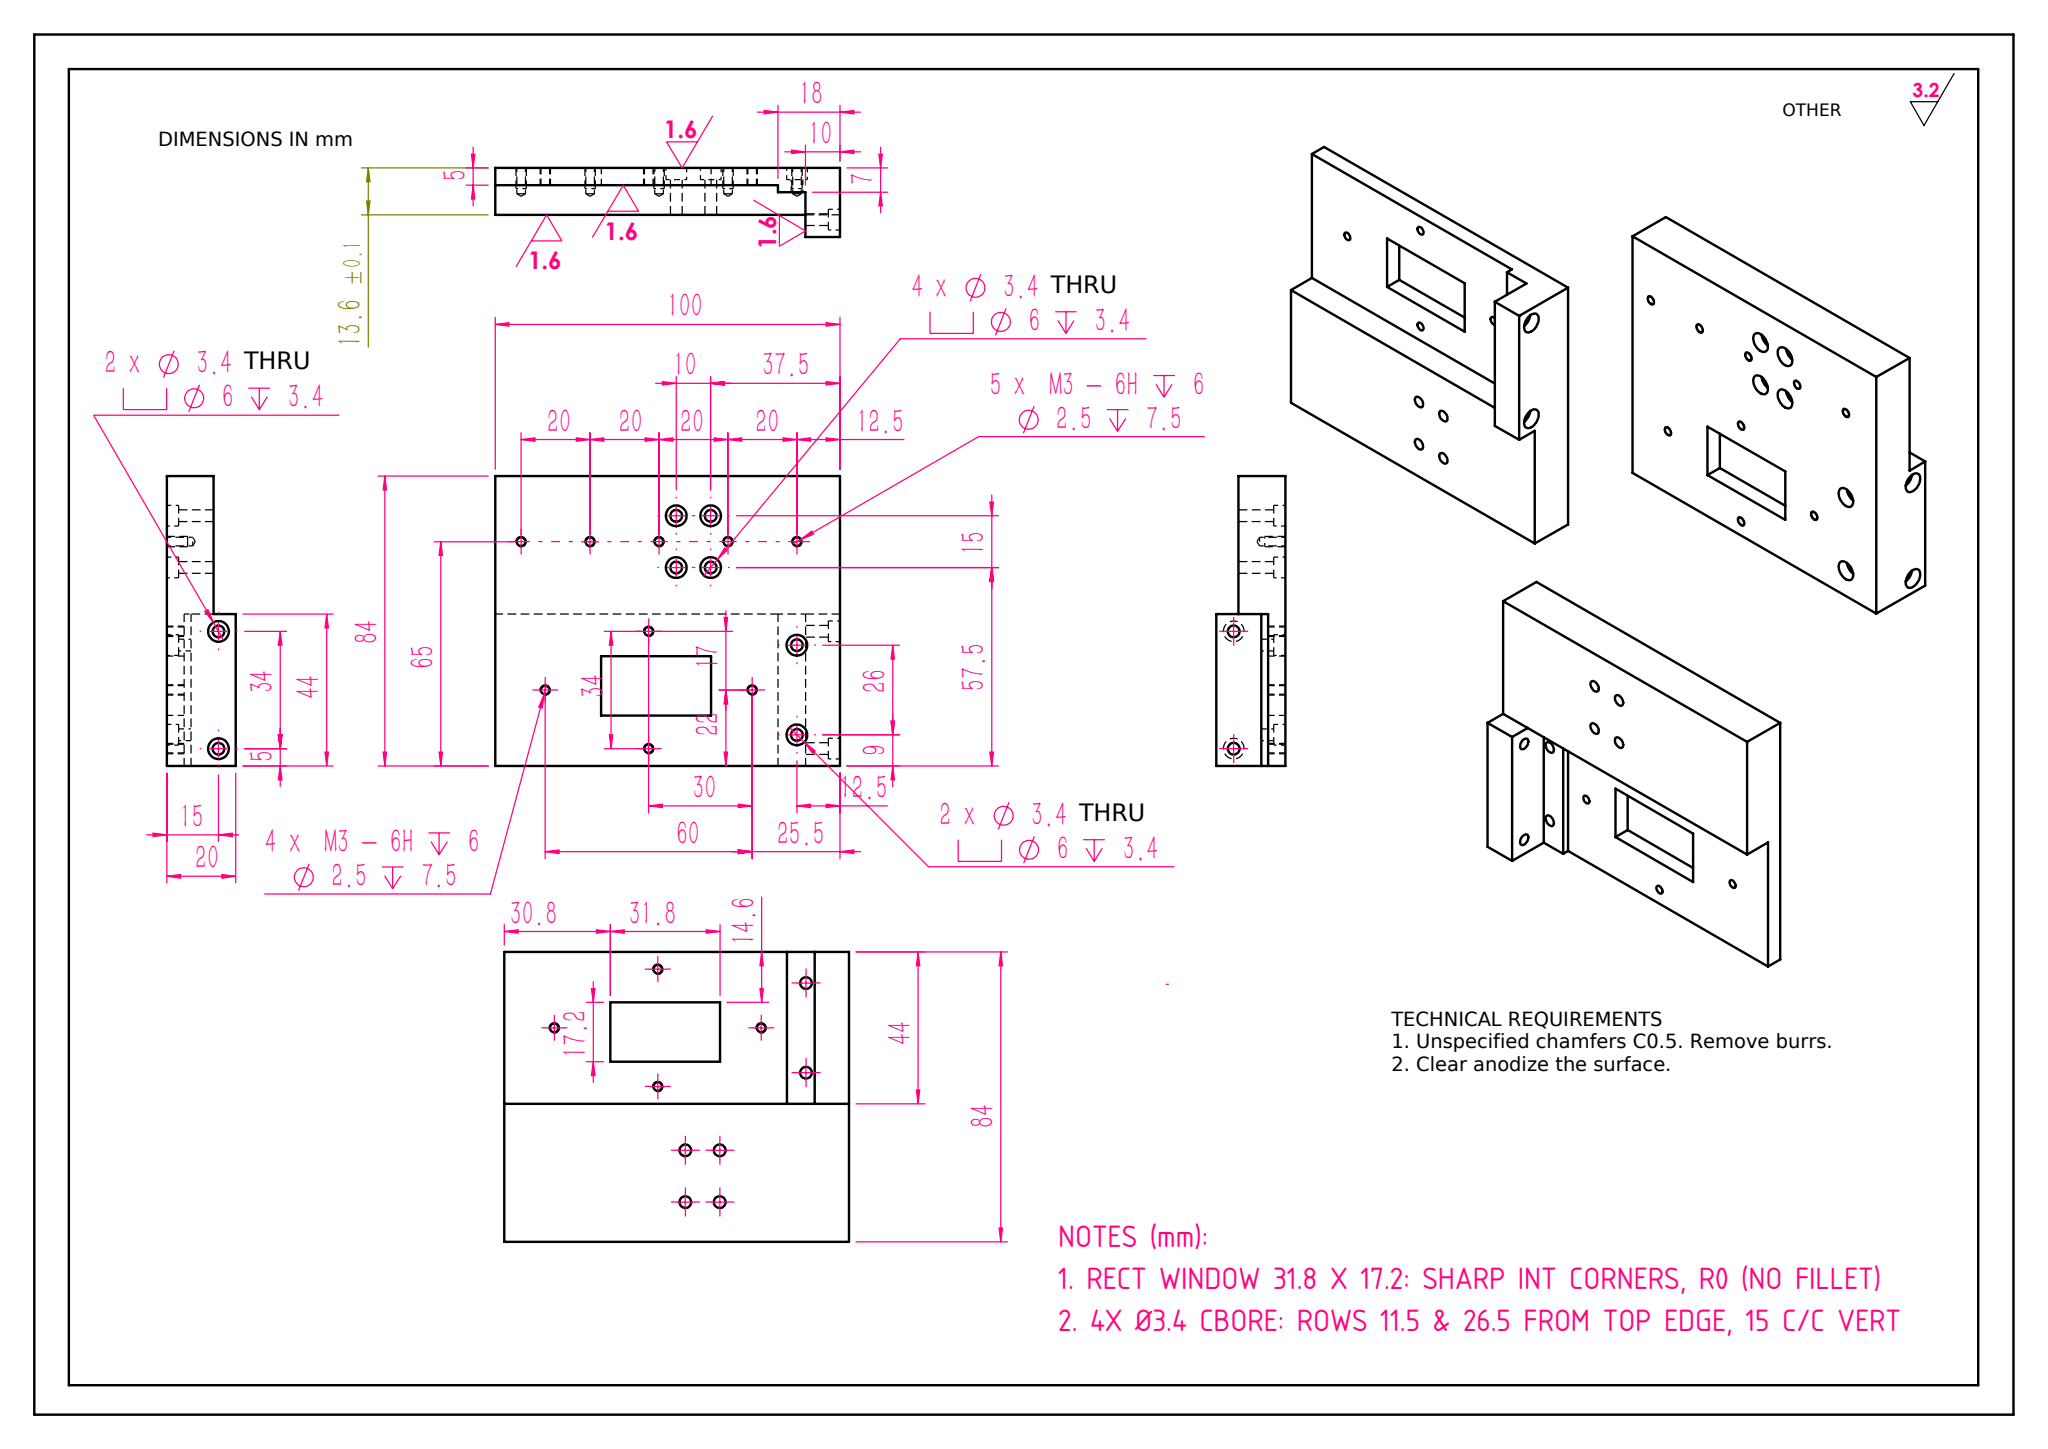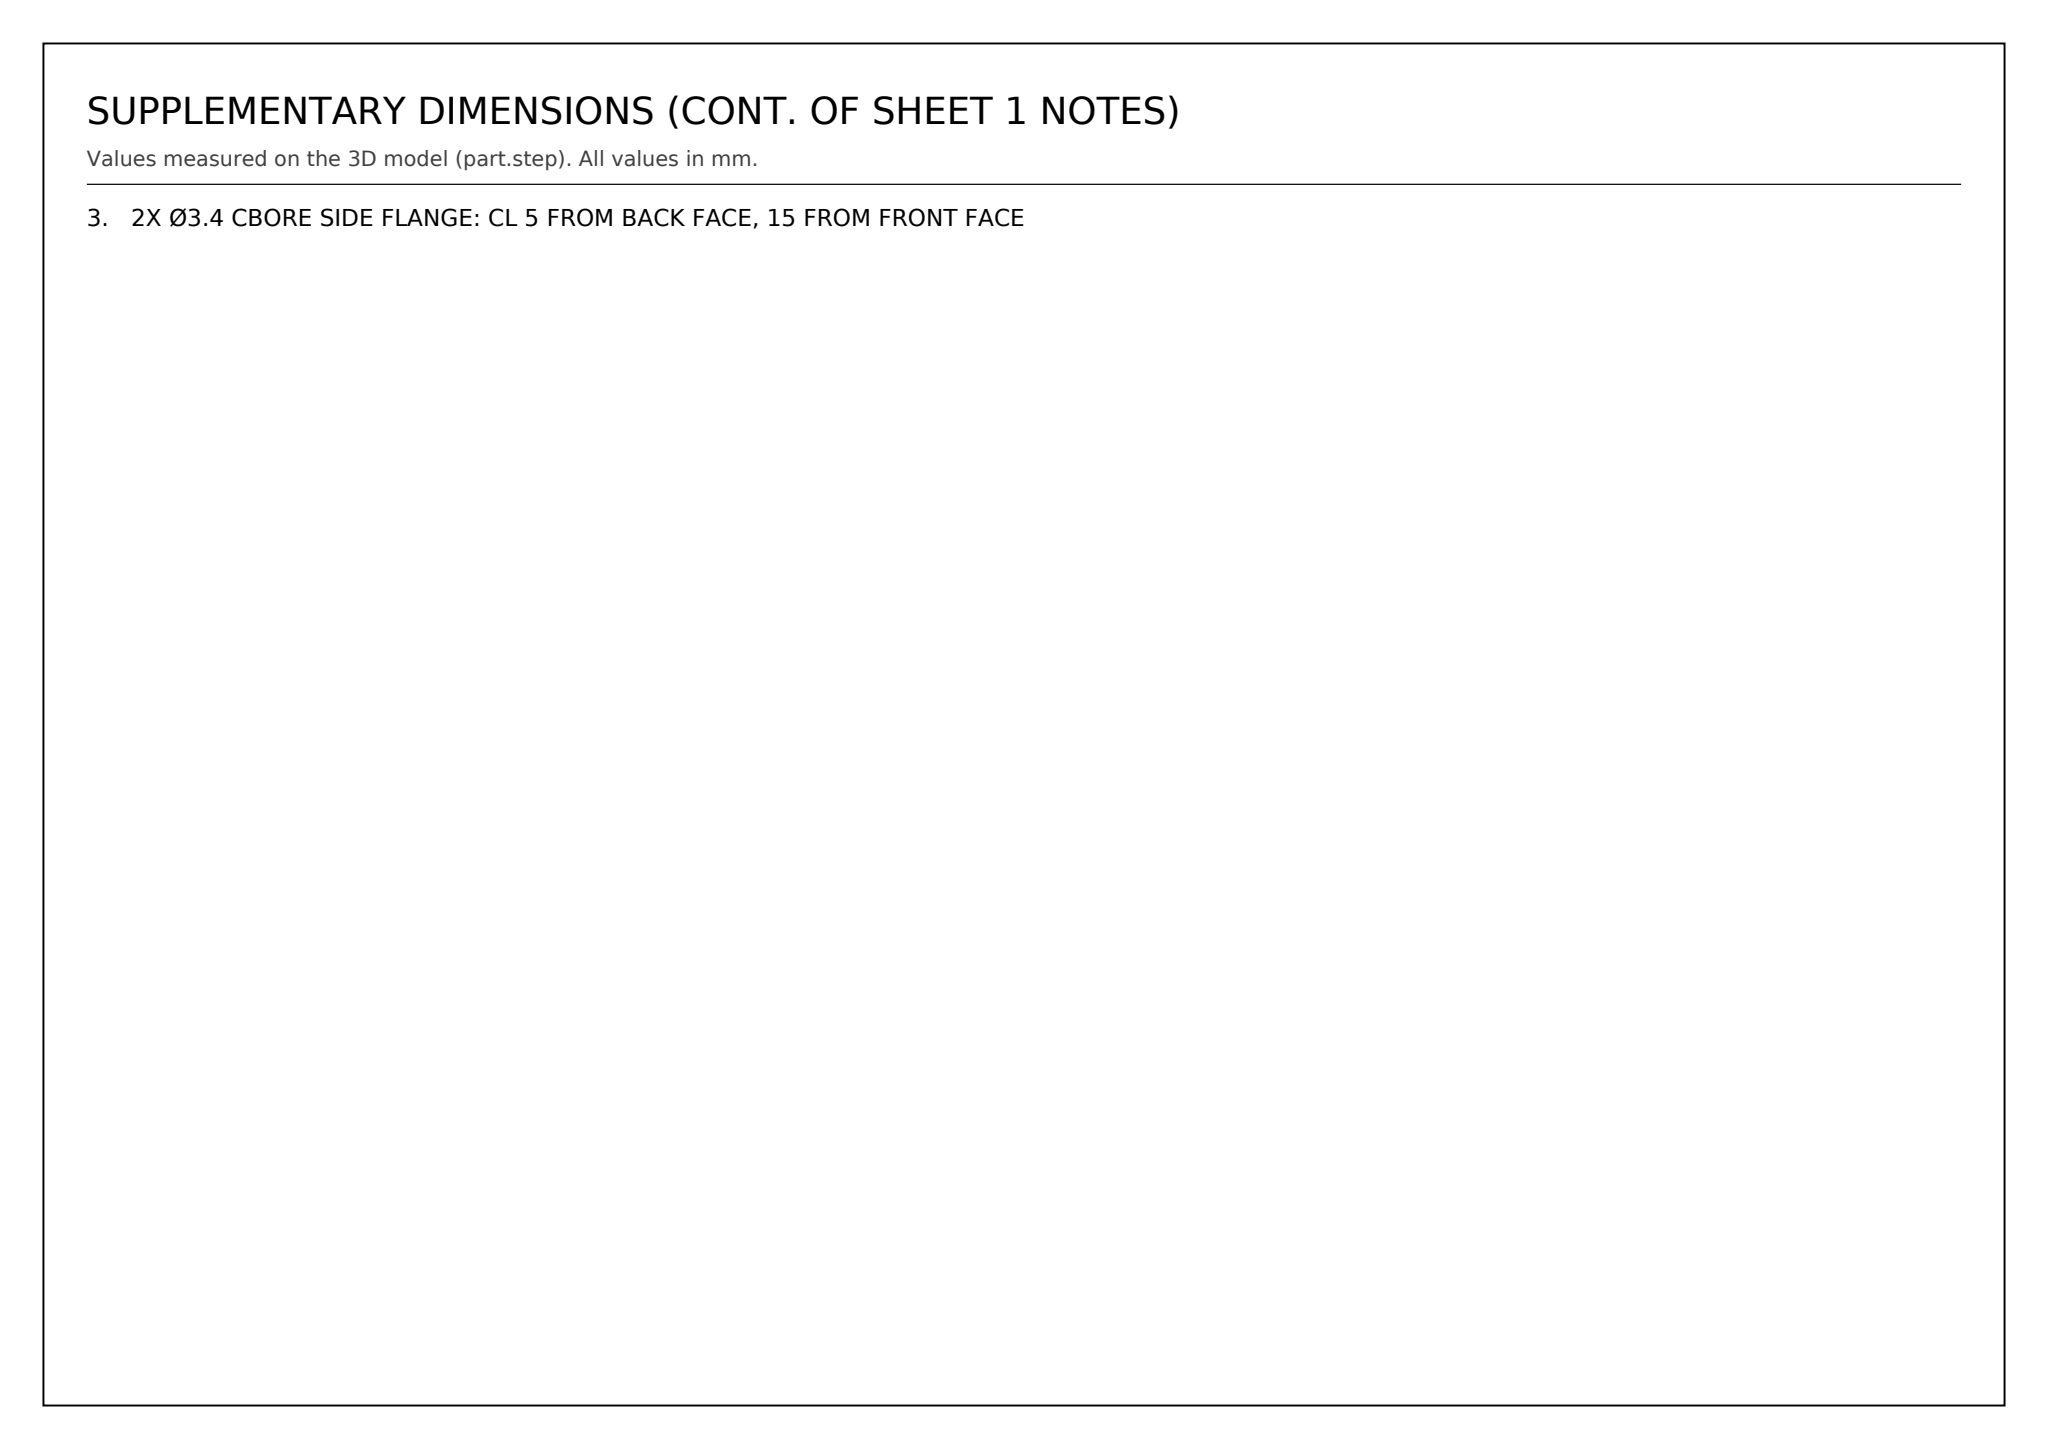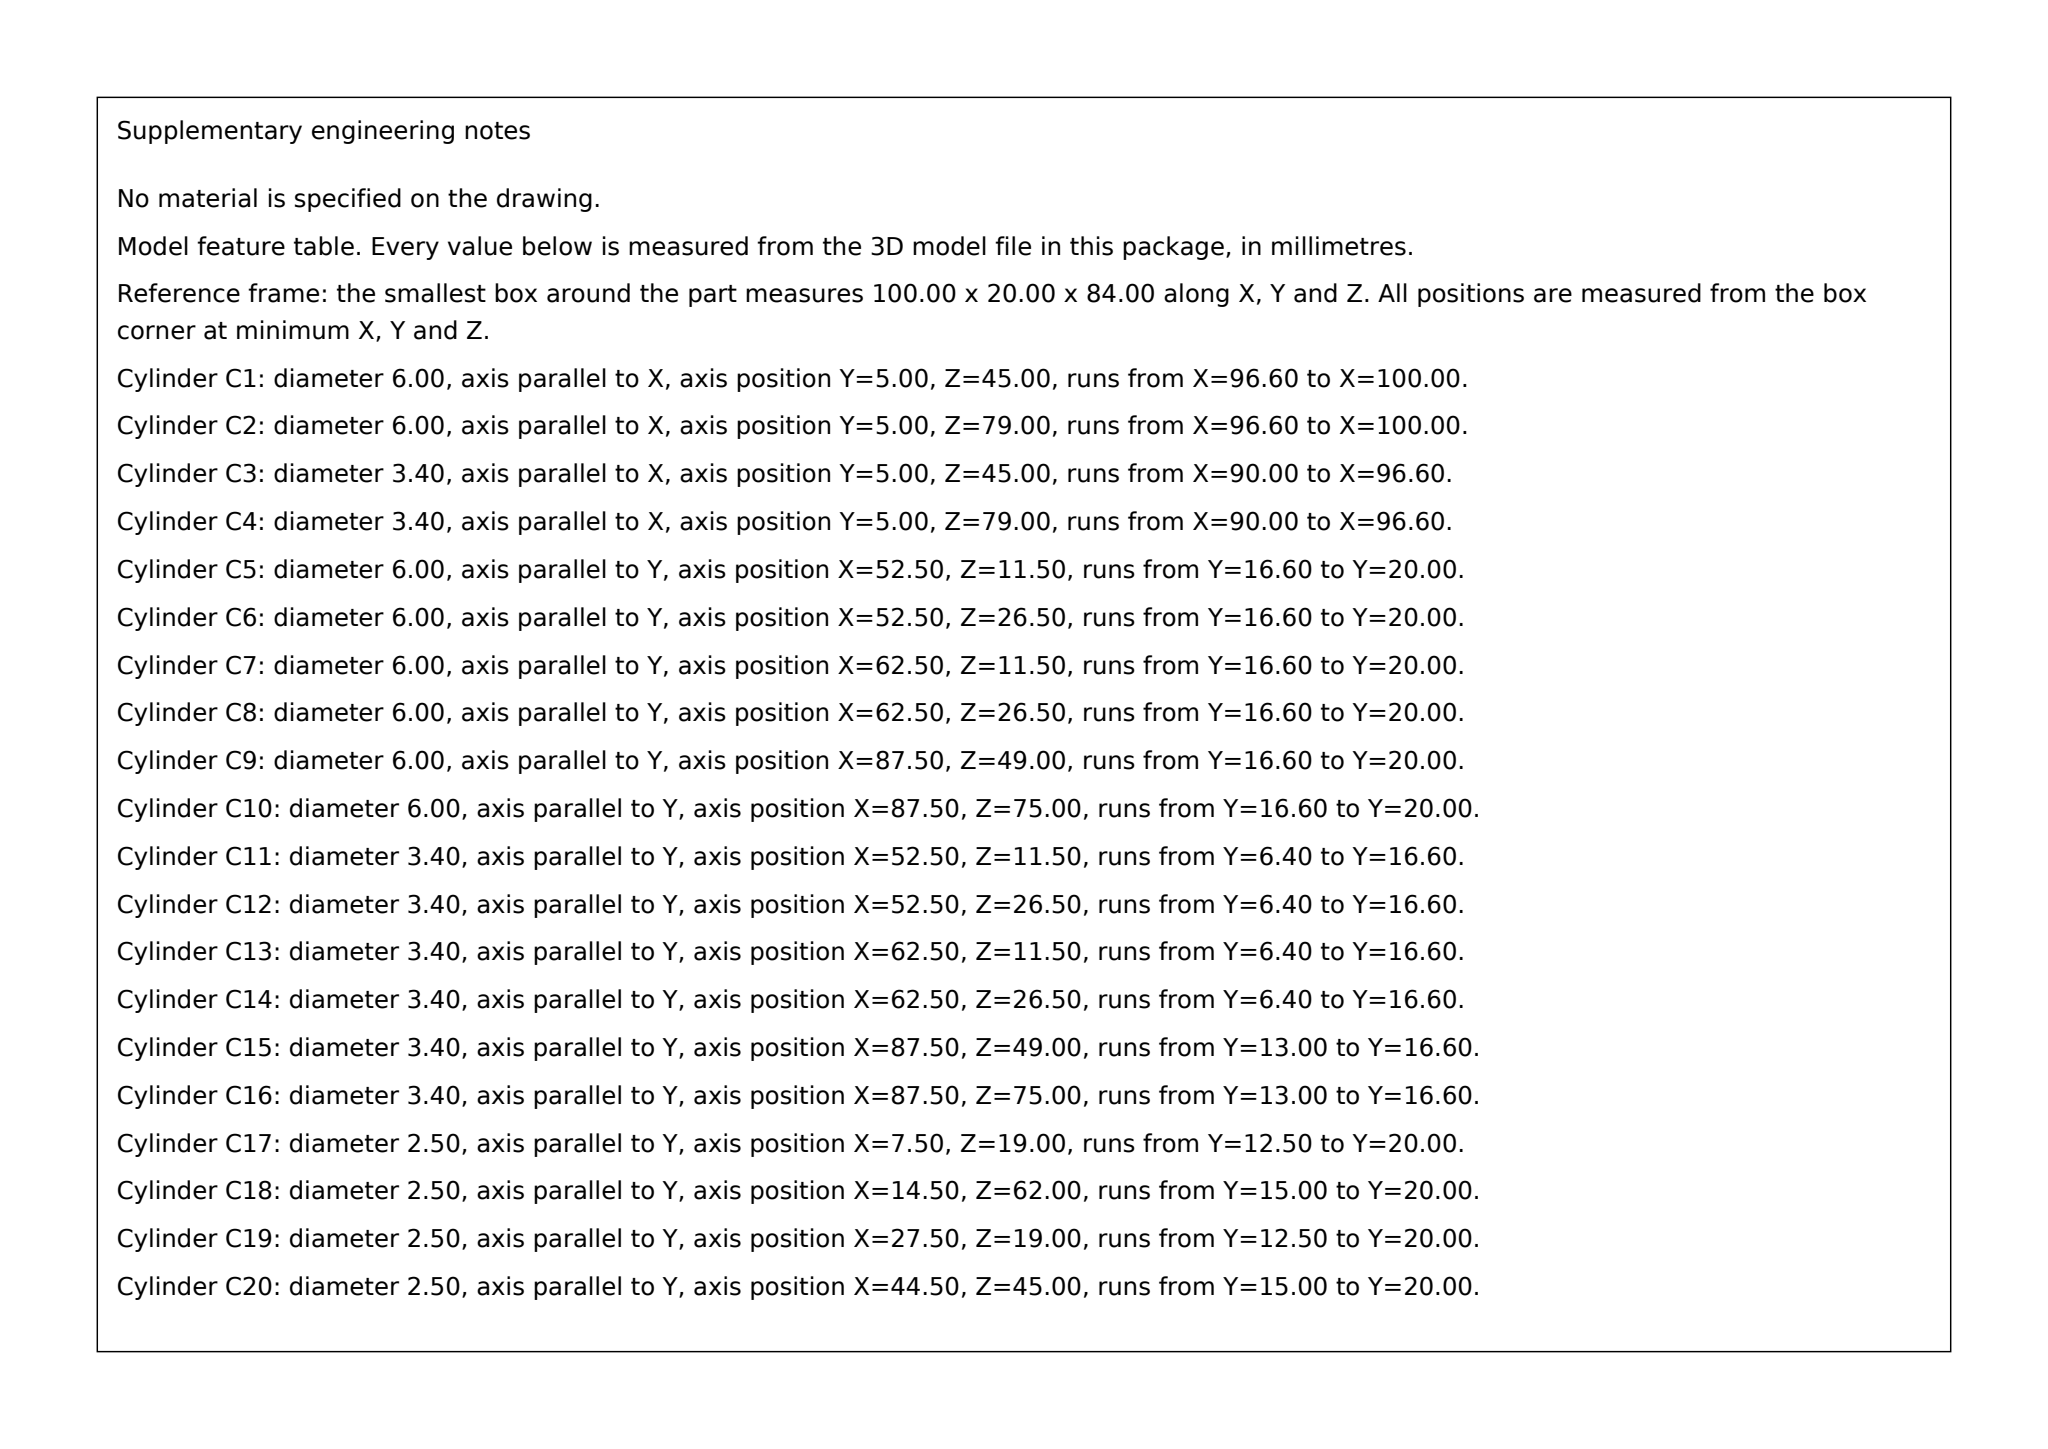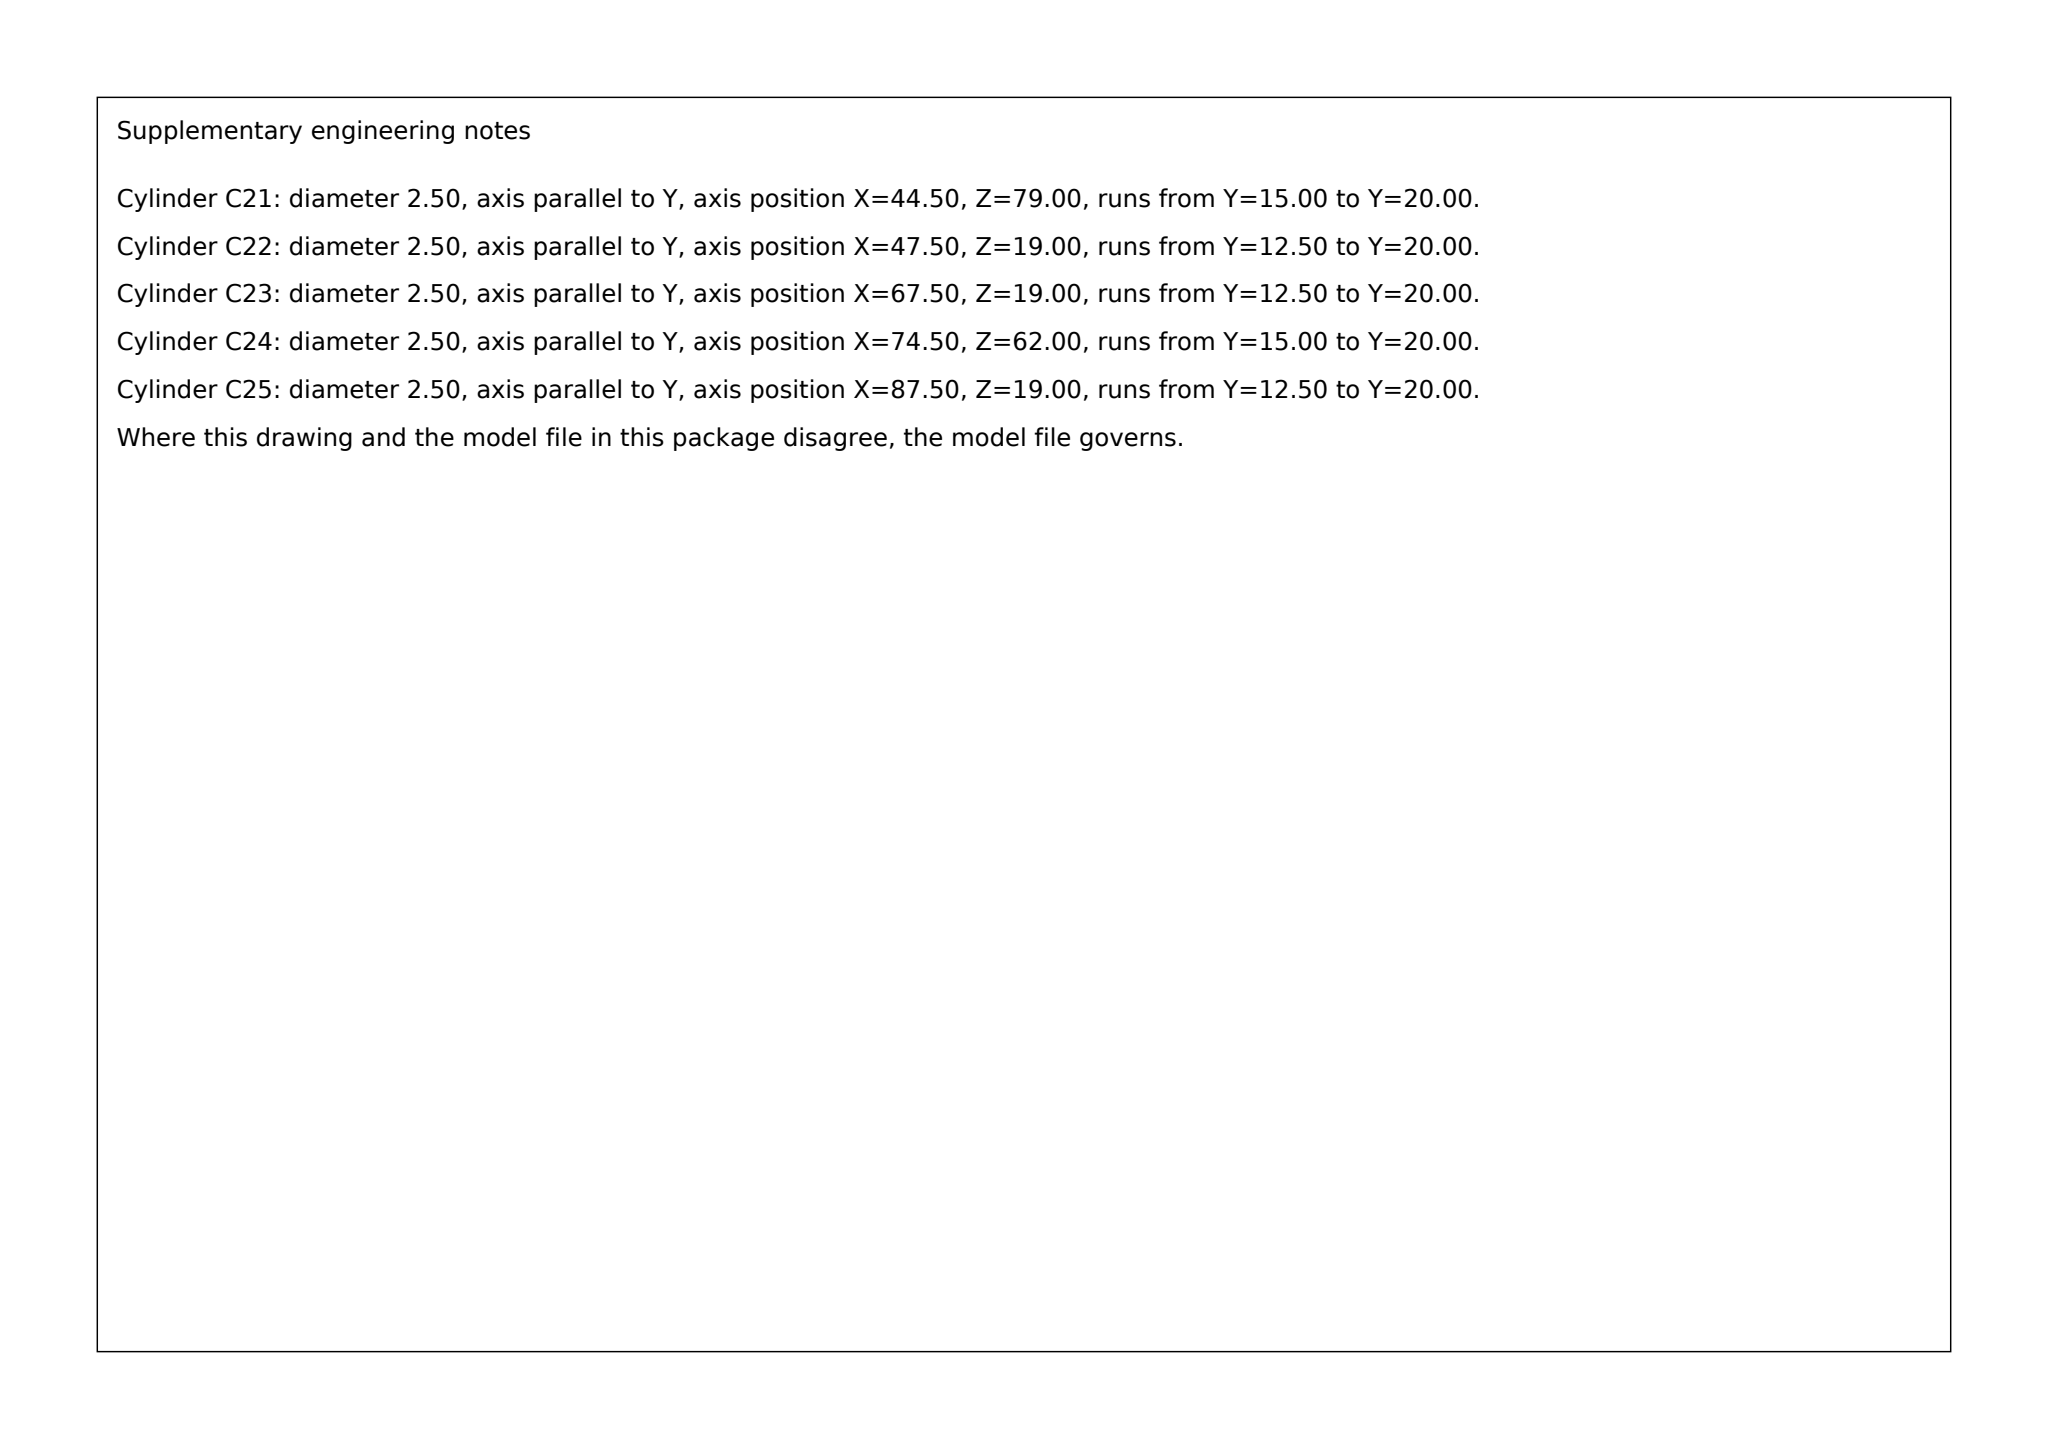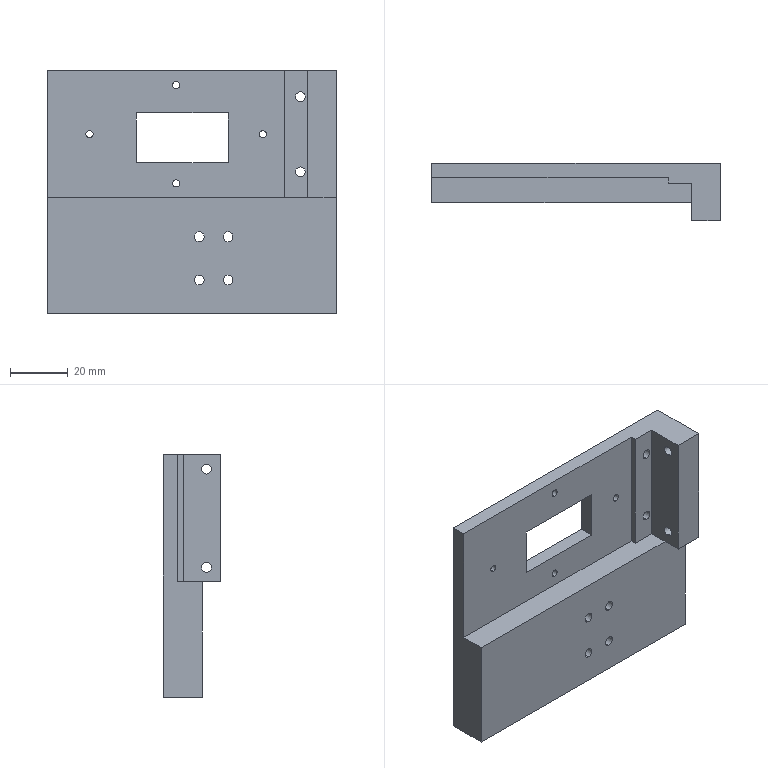Part | SolidWorks | mm | 1 solid | 85 faces | box 100 x 20 x 84 mm | volume 79353 mm3 | cylinder 50 | plane 25 | cone 10 | commonest cylinder face diameters 2.5 x18 6 x16 3.4 x16
Drawing notes:
RECT WINDOW 31.8 X 17.2: SHARP INT CORNERS, R0 (NO FILLET) | from the solid: fillet_radii: [] - pocket walls x=30.75/62.59, z=52.19/69.39 meet with no radius
4X Ø3.4 CBORE: ROWS 11.5 & 26.5 FROM TOP EDGE, 15 C/C VERT | from the solid: Ø3.4/Ø6 y-axis holes at z=11.5 and z=26.5 (x=52.5 & 62.5); 26.5-11.5=15; bbox z=84
2X Ø3.4 CBORE SIDE FLANGE: CL 5 FROM BACK FACE, 15 FROM FRONT FACE | from the solid: cylinders [3.4,x,[null,5.0,45.0]] & [3.4,x,[null,5.0,79.0]]; y planes 0 and 20 (20 wide flange) -> 5 / 15
build123d program:
from build123d import *

# Parameters (mm, degrees)
SKETCH1_W                                            = 100
SKETCH1_H                                            = 44
BOSS_EXTRUDE1_DEPTH                                  = 20
SKETCH2_W                                            = 90
SKETCH2_H                                            = 13
CUT_EXTRUDE1_DEPTH                                   = 70.541
SKETCH3_W                                            = 82
SKETCH3_H                                            = 2
CUT_EXTRUDE2_DEPTH                                   = 70.541
HOLE_SIZE_ACCORDING_TO_HEX_SOCKET_HEAD_C_D           = 3.4
HOLE_SIZE_ACCORDING_TO_HEX_SOCKET_HEAD_C_CBORE_D     = 6
HOLE_SIZE_ACCORDING_TO_HEX_SOCKET_HEAD_C_CBORE_DEPTH = 3.4
HOLE_SIZE_ACCORDING_TO_HEX_SOCKET_HE_2_D             = 3.4
HOLE_SIZE_ACCORDING_TO_HEX_SOCKET_HE_2_CBORE_D       = 6
HOLE_SIZE_ACCORDING_TO_HEX_SOCKET_HE_2_CBORE_DEPTH   = 3.4
M3_TAPPED_HOLE1_D                                    = 2.5
M3_TAPPED_HOLE1_DEPTH                                = 7.5
M3_TAPPED_HOLE1_TIP                                  = 0.7511
SKETCH11_W                                           = 100
SKETCH11_H                                           = 13.6
BOSS_EXTRUDE2_DEPTH                                  = 40
HOLE_SIZE_ACCORDING_TO_HEX_SOCKET_HE_3_D             = 3.4
HOLE_SIZE_ACCORDING_TO_HEX_SOCKET_HE_3_CBORE_D       = 6
HOLE_SIZE_ACCORDING_TO_HEX_SOCKET_HE_3_CBORE_DEPTH   = 3.4
LPATTERN1_COUNT                                      = 5
LPATTERN1_PITCH                                      = 20
SKETCH20_W                                           = 31.837
SKETCH20_H                                           = 17.198
CUT_EXTRUDE3_DEPTH                                   = 71


with BuildPart() as part:
    # Sketch1 → Boss-Extrude1 (new body)
    with BuildSketch(Plane(origin=(0, 0, 0), x_dir=(1, 0, 0), z_dir=(0, 1, 0))):
        Rectangle(SKETCH1_W, SKETCH1_H)
    extrude(amount=BOSS_EXTRUDE1_DEPTH)

    # Sketch2 → Cut-Extrude1 (cut, through all)
    with BuildSketch(Plane(origin=(0, 0, -22), x_dir=(-1, 0, 0), z_dir=(0, 0, -1))):
        with Locations((5, 6.5)):
            Rectangle(SKETCH2_W, SKETCH2_H)
    extrude(amount=-CUT_EXTRUDE1_DEPTH, mode=Mode.SUBTRACT)

    # Sketch3 → Cut-Extrude2 (cut, through all)
    with BuildSketch(Plane(origin=(0, 0, -22), x_dir=(-1, 0, 0), z_dir=(0, 0, -1))):
        with Locations((9, 14)):
            Rectangle(SKETCH3_W, SKETCH3_H)
    extrude(amount=-CUT_EXTRUDE2_DEPTH, mode=Mode.SUBTRACT)

    # Hole Size according to Hex Socket Head C (through all)
    with Locations(Plane(origin=(50, 0, 0), x_dir=(0, 0, -1), z_dir=(1, 0, 0))):
        with Locations((-17, 5), (17, 5)):
            CounterBoreHole(HOLE_SIZE_ACCORDING_TO_HEX_SOCKET_HEAD_C_D / 2, HOLE_SIZE_ACCORDING_TO_HEX_SOCKET_HEAD_C_CBORE_D / 2, HOLE_SIZE_ACCORDING_TO_HEX_SOCKET_HEAD_C_CBORE_DEPTH)

    # Hole Size according to Hex Socket He 2 (through all)
    with Locations(Plane(origin=(0, 20, 0), x_dir=(1, 0, 0), z_dir=(0, 1, 0))):
        with Locations((37.5, 13), (37.5, -13)):
            CounterBoreHole(HOLE_SIZE_ACCORDING_TO_HEX_SOCKET_HE_2_D / 2, HOLE_SIZE_ACCORDING_TO_HEX_SOCKET_HE_2_CBORE_D / 2, HOLE_SIZE_ACCORDING_TO_HEX_SOCKET_HE_2_CBORE_DEPTH)

    # M3 Tapped Hole1
    with Locations(Plane(origin=(0, 20, 0), x_dir=(1, 0, 0), z_dir=(0, 1, 0))):
        with Locations((24.5, 0), (-5.5, -17), (-5.5, 17), (-35.5, 0)):
            Hole(M3_TAPPED_HOLE1_D / 2, depth=M3_TAPPED_HOLE1_DEPTH)
            with Locations((0, 0, -(M3_TAPPED_HOLE1_DEPTH + M3_TAPPED_HOLE1_TIP / 2))):  # 118° drill point
                Cone(0, M3_TAPPED_HOLE1_D / 2, M3_TAPPED_HOLE1_TIP, mode=Mode.SUBTRACT)

    # Sketch11 → Boss-Extrude2 (add)
    with BuildSketch(Plane(origin=(0, 0, -22), x_dir=(-1, 0, 0), z_dir=(0, 0, -1))):
        with Locations((0, 13.2)):
            Rectangle(SKETCH11_W, SKETCH11_H)
    extrude(amount=BOSS_EXTRUDE2_DEPTH)

    # Hole Size according to Hex Socket He 3 (through all)
    with Locations(Plane(origin=(0, 20, 0), x_dir=(1, 0, 0), z_dir=(0, 1, 0))):
        with Locations((12.5, 50.5), (12.5, 35.5), (2.5, 50.5), (2.5, 35.5)):
            CounterBoreHole(HOLE_SIZE_ACCORDING_TO_HEX_SOCKET_HE_3_D / 2, HOLE_SIZE_ACCORDING_TO_HEX_SOCKET_HE_3_CBORE_D / 2, HOLE_SIZE_ACCORDING_TO_HEX_SOCKET_HE_3_CBORE_DEPTH)

    # Sketch18 → M3 Tapped Hole2 (revolve, cut)
    with BuildSketch(Plane(origin=(-42.5, 20, -43), x_dir=(0, 0, 1), z_dir=(1, 0, 0))):
        Polygon((0, 0), (0, 8.251), (1.25, 7.5), (1.25, 0), align=None)
    m3_tapped_hole2 = revolve(axis=Axis((-42.5, 26.35, -43), (0, -1, 0)), mode=Mode.SUBTRACT)

    # LPattern1: M3 Tapped Hole2 ×5
    with Locations(*[(i * LPATTERN1_PITCH, 0, 0) for i in range(1, LPATTERN1_COUNT)]):
        add(m3_tapped_hole2, mode=Mode.SUBTRACT)

    # Sketch20 → Cut-Extrude3 (cut)
    with BuildSketch(Plane.XZ.offset(-15)):
        with Locations((-3.327, -1.214)):
            Rectangle(SKETCH20_W, SKETCH20_H)
    extrude(amount=-CUT_EXTRUDE3_DEPTH, mode=Mode.SUBTRACT)


solid = part.part